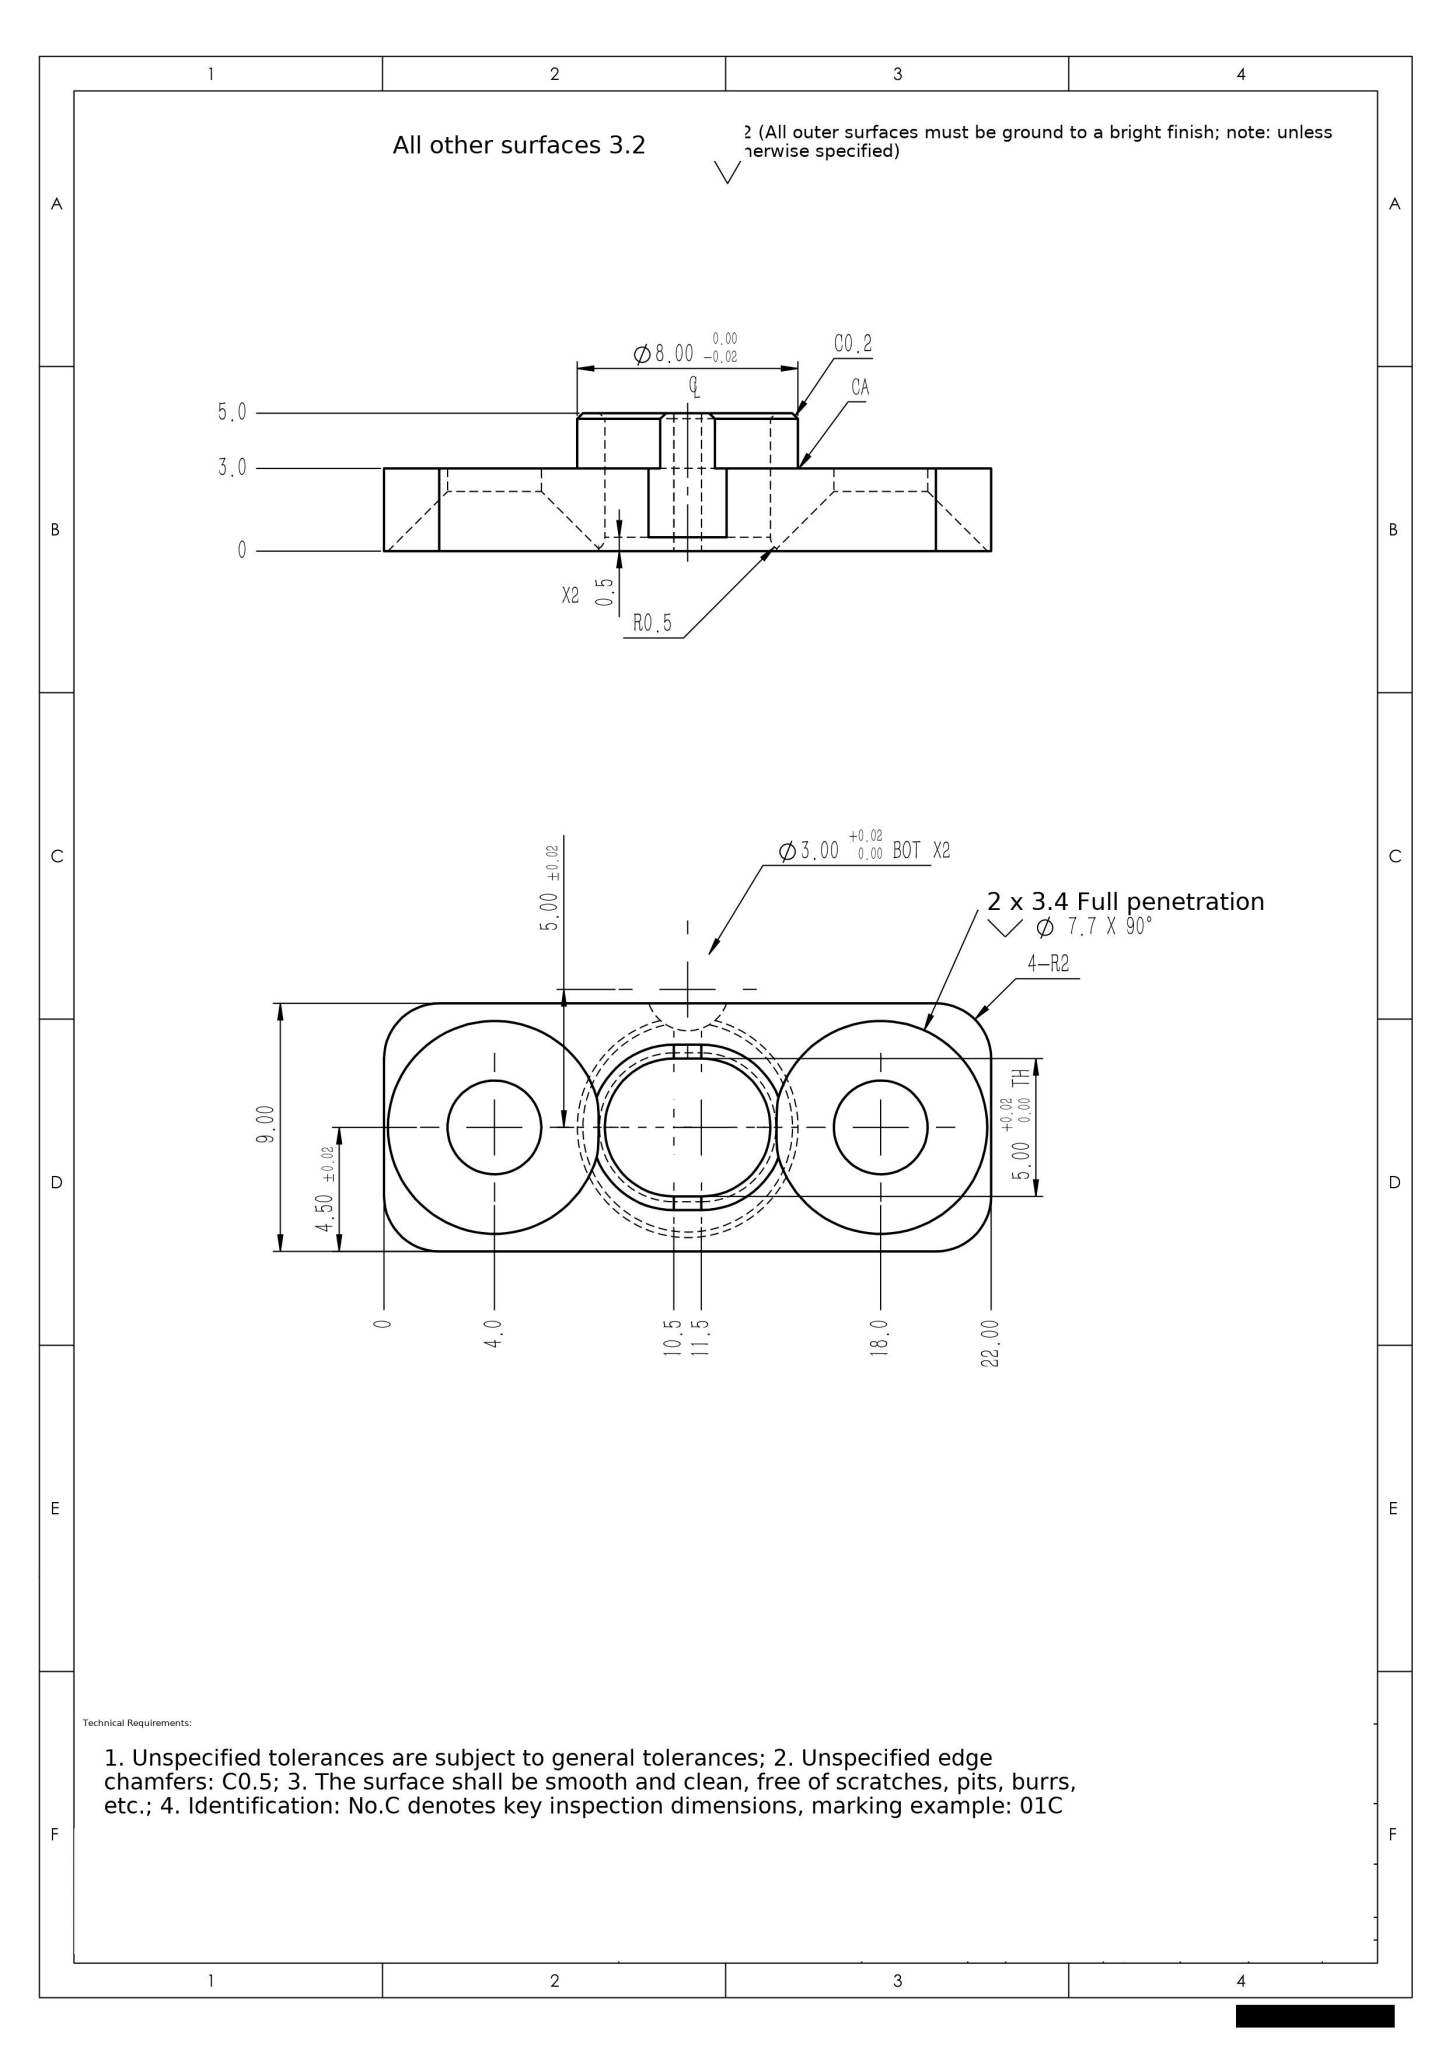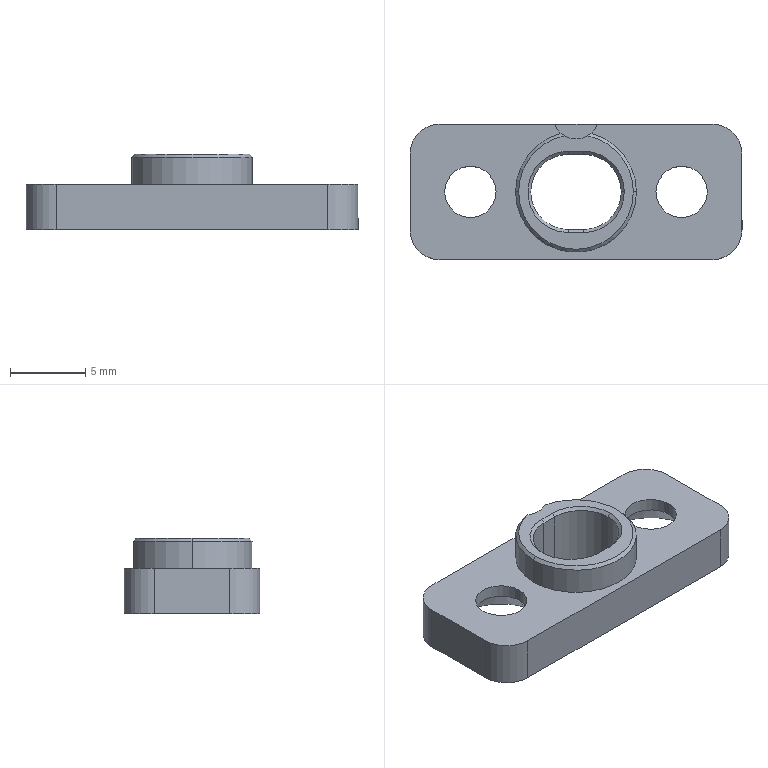Part | SolidWorks | mm | 1 solid | 42 faces | box 22 x 9 x 5 mm | volume 427 mm3 | cylinder 17 | plane 12 | cone 10 | torus 3 | commonest cylinder face diameters 3.4 x4 4 x4 5 x3 8 x3 1 x2 3 x1